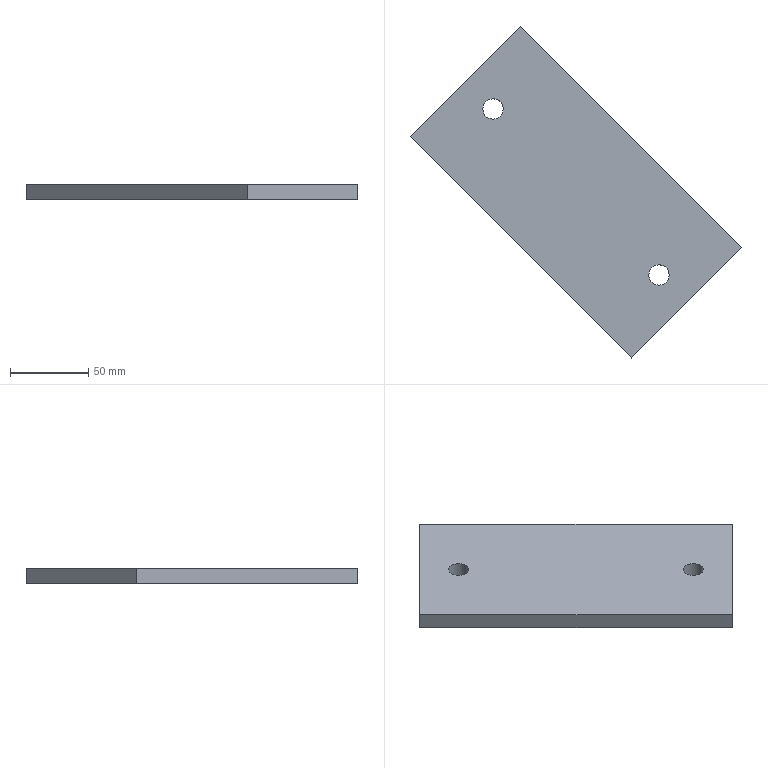Component | NX | CONN_FRAME_CONN_PLATE | 1 solid | 8 faces | box 212.13 x 212.13 x 10 mm | volume 197345 mm3 | plane 6 | cylinder 2 | commonest cylinder face diameters 13 x2
STEP:
#1=CARTESIAN_POINT('',(0.,0.,0.));
#2=DIRECTION('',(0.,0.,1.));
#3=DIRECTION('',(1.,0.,0.));
#4=AXIS2_PLACEMENT_3D('',#1,#2,#3);
#5=CARTESIAN_POINT('',(-344.075,421.231,520.));
#6=VERTEX_POINT('',#5);
#7=CARTESIAN_POINT('',(-202.653,279.81,520.));
#8=VERTEX_POINT('',#7);
#9=CARTESIAN_POINT('',(-344.075,421.231,520.));
#10=DIRECTION('',(0.7071,-0.7071,0.));
#11=VECTOR('',#10,1.);
#12=LINE('',#9,#11);
#13=CARTESIAN_POINT('',(-344.075,421.231,530.));
#14=DIRECTION('',(0.7071,0.7071,0.));
#15=DIRECTION('',(0.,0.,-1.));
#16=AXIS2_PLACEMENT_3D('',#13,#14,#15);
#17=PLANE('',#16);
#18=CARTESIAN_POINT('',(10.,0.));
#19=DIRECTION('',(0.,-1.));
#20=VECTOR('',#19,1.);
#21=LINE('',#18,#20);
#22=(GEOMETRIC_REPRESENTATION_CONTEXT(2)PARAMETRIC_REPRESENTATION_CONTEXT()REPRESENTATION_CONTEXT('',''));
#23=DEFINITIONAL_REPRESENTATION('',(#21),#22);
#24=PCURVE('',#17,#23);
#25=CARTESIAN_POINT('',(-361.752,368.198,520.));
#26=DIRECTION('',(0.,0.,1.));
#27=DIRECTION('',(-0.7071,0.7071,0.));
#28=AXIS2_PLACEMENT_3D('',#25,#26,#27);
#29=PLANE('',#28);
#30=CARTESIAN_POINT('',(25.,-50.));
#31=DIRECTION('',(-1.,0.));
#32=VECTOR('',#31,1.);
#33=LINE('',#30,#32);
#34=(GEOMETRIC_REPRESENTATION_CONTEXT(2)PARAMETRIC_REPRESENTATION_CONTEXT()REPRESENTATION_CONTEXT('',''));
#35=DEFINITIONAL_REPRESENTATION('',(#33),#34);
#36=PCURVE('',#29,#35);
#37=SURFACE_CURVE('',#12,(#24,#36),.PCURVE_S1.);
#38=EDGE_CURVE('',#6,#8,#37,.T.);
#39=ORIENTED_EDGE('',*,*,#38,.F.);
#40=CARTESIAN_POINT('',(-344.075,421.231,530.));
#41=VERTEX_POINT('',#40);
#42=CARTESIAN_POINT('',(-344.075,421.231,530.));
#43=DIRECTION('',(0.,0.,-1.));
#44=VECTOR('',#43,1.);
#45=LINE('',#42,#44);
#46=CARTESIAN_POINT('',(0.,0.));
#47=DIRECTION('',(1.,0.));
#48=VECTOR('',#47,1.);
#49=LINE('',#46,#48);
#50=(GEOMETRIC_REPRESENTATION_CONTEXT(2)PARAMETRIC_REPRESENTATION_CONTEXT()REPRESENTATION_CONTEXT('',''));
#51=DEFINITIONAL_REPRESENTATION('',(#49),#50);
#52=PCURVE('',#17,#51);
#53=CARTESIAN_POINT('',(-414.785,350.52,530.));
#54=DIRECTION('',(-0.7071,0.7071,0.));
#55=DIRECTION('',(0.,0.,-1.));
#56=AXIS2_PLACEMENT_3D('',#53,#54,#55);
#57=PLANE('',#56);
#58=CARTESIAN_POINT('',(0.,-100.));
#59=DIRECTION('',(1.,0.));
#60=VECTOR('',#59,1.);
#61=LINE('',#58,#60);
#62=(GEOMETRIC_REPRESENTATION_CONTEXT(2)PARAMETRIC_REPRESENTATION_CONTEXT()REPRESENTATION_CONTEXT('',''));
#63=DEFINITIONAL_REPRESENTATION('',(#61),#62);
#64=PCURVE('',#57,#63);
#65=SURFACE_CURVE('',#45,(#52,#64),.PCURVE_S1.);
#66=EDGE_CURVE('',#41,#6,#65,.T.);
#67=ORIENTED_EDGE('',*,*,#66,.F.);
#68=CARTESIAN_POINT('',(-202.653,279.81,530.));
#69=VERTEX_POINT('',#68);
#70=CARTESIAN_POINT('',(-344.075,421.231,530.));
#71=DIRECTION('',(0.7071,-0.7071,0.));
#72=VECTOR('',#71,1.);
#73=LINE('',#70,#72);
#74=CARTESIAN_POINT('',(0.,0.));
#75=DIRECTION('',(0.,-1.));
#76=VECTOR('',#75,1.);
#77=LINE('',#74,#76);
#78=(GEOMETRIC_REPRESENTATION_CONTEXT(2)PARAMETRIC_REPRESENTATION_CONTEXT()REPRESENTATION_CONTEXT('',''));
#79=DEFINITIONAL_REPRESENTATION('',(#77),#78);
#80=PCURVE('',#17,#79);
#81=CARTESIAN_POINT('',(-361.752,368.198,530.));
#82=DIRECTION('',(0.,0.,1.));
#83=DIRECTION('',(-0.7071,0.7071,0.));
#84=AXIS2_PLACEMENT_3D('',#81,#82,#83);
#85=PLANE('',#84);
#86=CARTESIAN_POINT('',(25.,-50.));
#87=DIRECTION('',(-1.,0.));
#88=VECTOR('',#87,1.);
#89=LINE('',#86,#88);
#90=(GEOMETRIC_REPRESENTATION_CONTEXT(2)PARAMETRIC_REPRESENTATION_CONTEXT()REPRESENTATION_CONTEXT('',''));
#91=DEFINITIONAL_REPRESENTATION('',(#89),#90);
#92=PCURVE('',#85,#91);
#93=SURFACE_CURVE('',#73,(#80,#92),.PCURVE_S1.);
#94=EDGE_CURVE('',#41,#69,#93,.T.);
#95=ORIENTED_EDGE('',*,*,#94,.T.);
#96=CARTESIAN_POINT('',(-202.653,279.81,530.));
#97=DIRECTION('',(0.,0.,-1.));
#98=VECTOR('',#97,1.);
#99=LINE('',#96,#98);
#100=CARTESIAN_POINT('',(0.,-200.));
#101=DIRECTION('',(1.,0.));
#102=VECTOR('',#101,1.);
#103=LINE('',#100,#102);
#104=(GEOMETRIC_REPRESENTATION_CONTEXT(2)PARAMETRIC_REPRESENTATION_CONTEXT()REPRESENTATION_CONTEXT('',''));
#105=DEFINITIONAL_REPRESENTATION('',(#103),#104);
#106=PCURVE('',#17,#105);
#107=CARTESIAN_POINT('',(-202.653,279.81,530.));
#108=DIRECTION('',(0.7071,-0.7071,0.));
#109=DIRECTION('',(0.,0.,1.));
#110=AXIS2_PLACEMENT_3D('',#107,#108,#109);
#111=PLANE('',#110);
#112=CARTESIAN_POINT('',(0.,0.));
#113=DIRECTION('',(-1.,0.));
#114=VECTOR('',#113,1.);
#115=LINE('',#112,#114);
#116=(GEOMETRIC_REPRESENTATION_CONTEXT(2)PARAMETRIC_REPRESENTATION_CONTEXT()REPRESENTATION_CONTEXT('',''));
#117=DEFINITIONAL_REPRESENTATION('',(#115),#116);
#118=PCURVE('',#111,#117);
#119=SURFACE_CURVE('',#99,(#106,#118),.PCURVE_S1.);
#120=EDGE_CURVE('',#69,#8,#119,.T.);
#121=ORIENTED_EDGE('',*,*,#120,.T.);
#122=EDGE_LOOP('',(#39,#67,#95,#121));
#123=FACE_BOUND('',#122,.T.);
#124=ADVANCED_FACE('',(#123),#17,.T.);
#125=CARTESIAN_POINT('',(-273.364,209.099,520.));
#126=VERTEX_POINT('',#125);
#127=CARTESIAN_POINT('',(-202.653,279.81,520.));
#128=DIRECTION('',(-0.7071,-0.7071,0.));
#129=VECTOR('',#128,1.);
#130=LINE('',#127,#129);
#131=CARTESIAN_POINT('',(-10.,0.));
#132=DIRECTION('',(0.,1.));
#133=VECTOR('',#132,1.);
#134=LINE('',#131,#133);
#135=(GEOMETRIC_REPRESENTATION_CONTEXT(2)PARAMETRIC_REPRESENTATION_CONTEXT()REPRESENTATION_CONTEXT('',''));
#136=DEFINITIONAL_REPRESENTATION('',(#134),#135);
#137=PCURVE('',#111,#136);
#138=CARTESIAN_POINT('',(-175.,-50.));
#139=DIRECTION('',(0.,1.));
#140=VECTOR('',#139,1.);
#141=LINE('',#138,#140);
#142=(GEOMETRIC_REPRESENTATION_CONTEXT(2)PARAMETRIC_REPRESENTATION_CONTEXT()REPRESENTATION_CONTEXT('',''));
#143=DEFINITIONAL_REPRESENTATION('',(#141),#142);
#144=PCURVE('',#29,#143);
#145=SURFACE_CURVE('',#130,(#137,#144),.PCURVE_S1.);
#146=EDGE_CURVE('',#8,#126,#145,.T.);
#147=ORIENTED_EDGE('',*,*,#146,.F.);
#148=ORIENTED_EDGE('',*,*,#120,.F.);
#149=CARTESIAN_POINT('',(-273.364,209.099,530.));
#150=VERTEX_POINT('',#149);
#151=CARTESIAN_POINT('',(-202.653,279.81,530.));
#152=DIRECTION('',(-0.7071,-0.7071,0.));
#153=VECTOR('',#152,1.);
#154=LINE('',#151,#153);
#155=CARTESIAN_POINT('',(0.,0.));
#156=DIRECTION('',(0.,1.));
#157=VECTOR('',#156,1.);
#158=LINE('',#155,#157);
#159=(GEOMETRIC_REPRESENTATION_CONTEXT(2)PARAMETRIC_REPRESENTATION_CONTEXT()REPRESENTATION_CONTEXT('',''));
#160=DEFINITIONAL_REPRESENTATION('',(#158),#159);
#161=PCURVE('',#111,#160);
#162=CARTESIAN_POINT('',(-175.,-50.));
#163=DIRECTION('',(0.,1.));
#164=VECTOR('',#163,1.);
#165=LINE('',#162,#164);
#166=(GEOMETRIC_REPRESENTATION_CONTEXT(2)PARAMETRIC_REPRESENTATION_CONTEXT()REPRESENTATION_CONTEXT('',''));
#167=DEFINITIONAL_REPRESENTATION('',(#165),#166);
#168=PCURVE('',#85,#167);
#169=SURFACE_CURVE('',#154,(#161,#168),.PCURVE_S1.);
#170=EDGE_CURVE('',#69,#150,#169,.T.);
#171=ORIENTED_EDGE('',*,*,#170,.T.);
#172=CARTESIAN_POINT('',(-273.364,209.099,530.));
#173=DIRECTION('',(0.,0.,-1.));
#174=VECTOR('',#173,1.);
#175=LINE('',#172,#174);
#176=CARTESIAN_POINT('',(0.,100.));
#177=DIRECTION('',(-1.,0.));
#178=VECTOR('',#177,1.);
#179=LINE('',#176,#178);
#180=(GEOMETRIC_REPRESENTATION_CONTEXT(2)PARAMETRIC_REPRESENTATION_CONTEXT()REPRESENTATION_CONTEXT('',''));
#181=DEFINITIONAL_REPRESENTATION('',(#179),#180);
#182=PCURVE('',#111,#181);
#183=CARTESIAN_POINT('',(-273.364,209.099,530.));
#184=DIRECTION('',(-0.7071,-0.7071,0.));
#185=DIRECTION('',(0.,0.,1.));
#186=AXIS2_PLACEMENT_3D('',#183,#184,#185);
#187=PLANE('',#186);
#188=CARTESIAN_POINT('',(0.,0.));
#189=DIRECTION('',(-1.,0.));
#190=VECTOR('',#189,1.);
#191=LINE('',#188,#190);
#192=(GEOMETRIC_REPRESENTATION_CONTEXT(2)PARAMETRIC_REPRESENTATION_CONTEXT()REPRESENTATION_CONTEXT('',''));
#193=DEFINITIONAL_REPRESENTATION('',(#191),#192);
#194=PCURVE('',#187,#193);
#195=SURFACE_CURVE('',#175,(#182,#194),.PCURVE_S1.);
#196=EDGE_CURVE('',#150,#126,#195,.T.);
#197=ORIENTED_EDGE('',*,*,#196,.T.);
#198=EDGE_LOOP('',(#147,#148,#171,#197));
#199=FACE_BOUND('',#198,.T.);
#200=ADVANCED_FACE('',(#199),#111,.T.);
#201=CARTESIAN_POINT('',(-414.785,350.52,520.));
#202=VERTEX_POINT('',#201);
#203=CARTESIAN_POINT('',(-273.364,209.099,520.));
#204=DIRECTION('',(-0.7071,0.7071,0.));
#205=VECTOR('',#204,1.);
#206=LINE('',#203,#205);
#207=CARTESIAN_POINT('',(-10.,0.));
#208=DIRECTION('',(0.,1.));
#209=VECTOR('',#208,1.);
#210=LINE('',#207,#209);
#211=(GEOMETRIC_REPRESENTATION_CONTEXT(2)PARAMETRIC_REPRESENTATION_CONTEXT()REPRESENTATION_CONTEXT('',''));
#212=DEFINITIONAL_REPRESENTATION('',(#210),#211);
#213=PCURVE('',#187,#212);
#214=CARTESIAN_POINT('',(-175.,50.));
#215=DIRECTION('',(1.,0.));
#216=VECTOR('',#215,1.);
#217=LINE('',#214,#216);
#218=(GEOMETRIC_REPRESENTATION_CONTEXT(2)PARAMETRIC_REPRESENTATION_CONTEXT()REPRESENTATION_CONTEXT('',''));
#219=DEFINITIONAL_REPRESENTATION('',(#217),#218);
#220=PCURVE('',#29,#219);
#221=SURFACE_CURVE('',#206,(#213,#220),.PCURVE_S1.);
#222=EDGE_CURVE('',#126,#202,#221,.T.);
#223=ORIENTED_EDGE('',*,*,#222,.F.);
#224=ORIENTED_EDGE('',*,*,#196,.F.);
#225=CARTESIAN_POINT('',(-414.785,350.52,530.));
#226=VERTEX_POINT('',#225);
#227=CARTESIAN_POINT('',(-273.364,209.099,530.));
#228=DIRECTION('',(-0.7071,0.7071,0.));
#229=VECTOR('',#228,1.);
#230=LINE('',#227,#229);
#231=CARTESIAN_POINT('',(0.,0.));
#232=DIRECTION('',(0.,1.));
#233=VECTOR('',#232,1.);
#234=LINE('',#231,#233);
#235=(GEOMETRIC_REPRESENTATION_CONTEXT(2)PARAMETRIC_REPRESENTATION_CONTEXT()REPRESENTATION_CONTEXT('',''));
#236=DEFINITIONAL_REPRESENTATION('',(#234),#235);
#237=PCURVE('',#187,#236);
#238=CARTESIAN_POINT('',(-175.,50.));
#239=DIRECTION('',(1.,0.));
#240=VECTOR('',#239,1.);
#241=LINE('',#238,#240);
#242=(GEOMETRIC_REPRESENTATION_CONTEXT(2)PARAMETRIC_REPRESENTATION_CONTEXT()REPRESENTATION_CONTEXT('',''));
#243=DEFINITIONAL_REPRESENTATION('',(#241),#242);
#244=PCURVE('',#85,#243);
#245=SURFACE_CURVE('',#230,(#237,#244),.PCURVE_S1.);
#246=EDGE_CURVE('',#150,#226,#245,.T.);
#247=ORIENTED_EDGE('',*,*,#246,.T.);
#248=CARTESIAN_POINT('',(-414.785,350.52,530.));
#249=DIRECTION('',(0.,0.,-1.));
#250=VECTOR('',#249,1.);
#251=LINE('',#248,#250);
#252=CARTESIAN_POINT('',(0.,200.));
#253=DIRECTION('',(-1.,0.));
#254=VECTOR('',#253,1.);
#255=LINE('',#252,#254);
#256=(GEOMETRIC_REPRESENTATION_CONTEXT(2)PARAMETRIC_REPRESENTATION_CONTEXT()REPRESENTATION_CONTEXT('',''));
#257=DEFINITIONAL_REPRESENTATION('',(#255),#256);
#258=PCURVE('',#187,#257);
#259=CARTESIAN_POINT('',(0.,0.));
#260=DIRECTION('',(1.,0.));
#261=VECTOR('',#260,1.);
#262=LINE('',#259,#261);
#263=(GEOMETRIC_REPRESENTATION_CONTEXT(2)PARAMETRIC_REPRESENTATION_CONTEXT()REPRESENTATION_CONTEXT('',''));
#264=DEFINITIONAL_REPRESENTATION('',(#262),#263);
#265=PCURVE('',#57,#264);
#266=SURFACE_CURVE('',#251,(#258,#265),.PCURVE_S1.);
#267=EDGE_CURVE('',#226,#202,#266,.T.);
#268=ORIENTED_EDGE('',*,*,#267,.T.);
#269=EDGE_LOOP('',(#223,#224,#247,#268));
#270=FACE_BOUND('',#269,.T.);
#271=ADVANCED_FACE('',(#270),#187,.T.);
#272=CARTESIAN_POINT('',(-357.156,363.602,530.));
#273=VERTEX_POINT('',#272);
#274=CARTESIAN_POINT('',(-361.752,368.198,530.));
#275=DIRECTION('',(0.,0.,1.));
#276=DIRECTION('',(0.7071,-0.7071,0.));
#277=AXIS2_PLACEMENT_3D('',#274,#275,#276);
#278=CIRCLE('',#277,6.5);
#279=CARTESIAN_POINT('',(-361.752,368.198,530.));
#280=DIRECTION('',(0.,0.,-1.));
#281=DIRECTION('',(0.7071,-0.7071,0.));
#282=AXIS2_PLACEMENT_3D('',#279,#280,#281);
#283=CYLINDRICAL_SURFACE('',#282,6.5);
#284=CARTESIAN_POINT('',(6.283,0.));
#285=DIRECTION('',(-1.,0.));
#286=VECTOR('',#285,1.);
#287=LINE('',#284,#286);
#288=(GEOMETRIC_REPRESENTATION_CONTEXT(2)PARAMETRIC_REPRESENTATION_CONTEXT()REPRESENTATION_CONTEXT('',''));
#289=DEFINITIONAL_REPRESENTATION('',(#287),#288);
#290=PCURVE('',#283,#289);
#291=CARTESIAN_POINT('',(0.,0.));
#292=DIRECTION('',(-1.,-0.));
#293=AXIS2_PLACEMENT_2D('',#291,#292);
#294=CIRCLE('',#293,6.5);
#295=(GEOMETRIC_REPRESENTATION_CONTEXT(2)PARAMETRIC_REPRESENTATION_CONTEXT()REPRESENTATION_CONTEXT('',''));
#296=DEFINITIONAL_REPRESENTATION('',(#294),#295);
#297=PCURVE('',#85,#296);
#298=SURFACE_CURVE('',#278,(#290,#297),.PCURVE_S1.);
#299=EDGE_CURVE('',#273,#273,#298,.T.);
#300=ORIENTED_EDGE('',*,*,#299,.F.);
#301=CARTESIAN_POINT('',(-357.156,363.602,520.));
#302=VERTEX_POINT('',#301);
#303=CARTESIAN_POINT('',(-357.156,363.602,530.));
#304=CARTESIAN_POINT('',(-357.156,363.602,520.));
#305=B_SPLINE_CURVE_WITH_KNOTS('',1,(#303,#304),.UNSPECIFIED.,.F.,.F.,(2,2),(0.,10.),.PIECEWISE_BEZIER_KNOTS.);
#306=CARTESIAN_POINT('',(6.283,0.));
#307=DIRECTION('',(0.,1.));
#308=VECTOR('',#307,1.);
#309=LINE('',#306,#308);
#310=(GEOMETRIC_REPRESENTATION_CONTEXT(2)PARAMETRIC_REPRESENTATION_CONTEXT()REPRESENTATION_CONTEXT('',''));
#311=DEFINITIONAL_REPRESENTATION('',(#309),#310);
#312=PCURVE('',#283,#311);
#313=CARTESIAN_POINT('',(0.,0.));
#314=DIRECTION('',(0.,1.));
#315=VECTOR('',#314,1.);
#316=LINE('',#313,#315);
#317=(GEOMETRIC_REPRESENTATION_CONTEXT(2)PARAMETRIC_REPRESENTATION_CONTEXT()REPRESENTATION_CONTEXT('',''));
#318=DEFINITIONAL_REPRESENTATION('',(#316),#317);
#319=PCURVE('',#283,#318);
#320=SEAM_CURVE('',#305,(#312,#319),.PCURVE_S1.);
#321=EDGE_CURVE('',#273,#302,#320,.T.);
#322=ORIENTED_EDGE('',*,*,#321,.T.);
#323=CARTESIAN_POINT('',(-361.752,368.198,520.));
#324=DIRECTION('',(0.,0.,1.));
#325=DIRECTION('',(0.7071,-0.7071,0.));
#326=AXIS2_PLACEMENT_3D('',#323,#324,#325);
#327=CIRCLE('',#326,6.5);
#328=CARTESIAN_POINT('',(6.283,10.));
#329=DIRECTION('',(-1.,0.));
#330=VECTOR('',#329,1.);
#331=LINE('',#328,#330);
#332=(GEOMETRIC_REPRESENTATION_CONTEXT(2)PARAMETRIC_REPRESENTATION_CONTEXT()REPRESENTATION_CONTEXT('',''));
#333=DEFINITIONAL_REPRESENTATION('',(#331),#332);
#334=PCURVE('',#283,#333);
#335=CARTESIAN_POINT('',(0.,0.));
#336=DIRECTION('',(-1.,-0.));
#337=AXIS2_PLACEMENT_2D('',#335,#336);
#338=CIRCLE('',#337,6.5);
#339=(GEOMETRIC_REPRESENTATION_CONTEXT(2)PARAMETRIC_REPRESENTATION_CONTEXT()REPRESENTATION_CONTEXT('',''));
#340=DEFINITIONAL_REPRESENTATION('',(#338),#339);
#341=PCURVE('',#29,#340);
#342=SURFACE_CURVE('',#327,(#334,#341),.PCURVE_S1.);
#343=EDGE_CURVE('',#302,#302,#342,.T.);
#344=ORIENTED_EDGE('',*,*,#343,.T.);
#345=ORIENTED_EDGE('',*,*,#321,.F.);
#346=EDGE_LOOP('',(#300,#322,#344,#345));
#347=FACE_BOUND('',#346,.F.);
#348=ADVANCED_FACE('',(#347),#283,.F.);
#349=CARTESIAN_POINT('',(-414.785,350.52,520.));
#350=DIRECTION('',(0.7071,0.7071,0.));
#351=VECTOR('',#350,1.);
#352=LINE('',#349,#351);
#353=CARTESIAN_POINT('',(10.,0.));
#354=DIRECTION('',(0.,-1.));
#355=VECTOR('',#354,1.);
#356=LINE('',#353,#355);
#357=(GEOMETRIC_REPRESENTATION_CONTEXT(2)PARAMETRIC_REPRESENTATION_CONTEXT()REPRESENTATION_CONTEXT('',''));
#358=DEFINITIONAL_REPRESENTATION('',(#356),#357);
#359=PCURVE('',#57,#358);
#360=CARTESIAN_POINT('',(25.,50.));
#361=DIRECTION('',(0.,-1.));
#362=VECTOR('',#361,1.);
#363=LINE('',#360,#362);
#364=(GEOMETRIC_REPRESENTATION_CONTEXT(2)PARAMETRIC_REPRESENTATION_CONTEXT()REPRESENTATION_CONTEXT('',''));
#365=DEFINITIONAL_REPRESENTATION('',(#363),#364);
#366=PCURVE('',#29,#365);
#367=SURFACE_CURVE('',#352,(#359,#366),.PCURVE_S1.);
#368=EDGE_CURVE('',#202,#6,#367,.T.);
#369=ORIENTED_EDGE('',*,*,#368,.F.);
#370=ORIENTED_EDGE('',*,*,#267,.F.);
#371=CARTESIAN_POINT('',(-414.785,350.52,530.));
#372=DIRECTION('',(0.7071,0.7071,0.));
#373=VECTOR('',#372,1.);
#374=LINE('',#371,#373);
#375=CARTESIAN_POINT('',(0.,0.));
#376=DIRECTION('',(0.,-1.));
#377=VECTOR('',#376,1.);
#378=LINE('',#375,#377);
#379=(GEOMETRIC_REPRESENTATION_CONTEXT(2)PARAMETRIC_REPRESENTATION_CONTEXT()REPRESENTATION_CONTEXT('',''));
#380=DEFINITIONAL_REPRESENTATION('',(#378),#379);
#381=PCURVE('',#57,#380);
#382=CARTESIAN_POINT('',(25.,50.));
#383=DIRECTION('',(0.,-1.));
#384=VECTOR('',#383,1.);
#385=LINE('',#382,#384);
#386=(GEOMETRIC_REPRESENTATION_CONTEXT(2)PARAMETRIC_REPRESENTATION_CONTEXT()REPRESENTATION_CONTEXT('',''));
#387=DEFINITIONAL_REPRESENTATION('',(#385),#386);
#388=PCURVE('',#85,#387);
#389=SURFACE_CURVE('',#374,(#381,#388),.PCURVE_S1.);
#390=EDGE_CURVE('',#226,#41,#389,.T.);
#391=ORIENTED_EDGE('',*,*,#390,.T.);
#392=ORIENTED_EDGE('',*,*,#66,.T.);
#393=EDGE_LOOP('',(#369,#370,#391,#392));
#394=FACE_BOUND('',#393,.T.);
#395=ADVANCED_FACE('',(#394),#57,.T.);
#396=CARTESIAN_POINT('',(-260.283,266.728,530.));
#397=VERTEX_POINT('',#396);
#398=CARTESIAN_POINT('',(-255.686,262.132,530.));
#399=DIRECTION('',(0.,0.,-1.));
#400=DIRECTION('',(-0.7071,0.7071,0.));
#401=AXIS2_PLACEMENT_3D('',#398,#399,#400);
#402=CIRCLE('',#401,6.5);
#403=CARTESIAN_POINT('',(-255.686,262.132,530.));
#404=DIRECTION('',(0.,0.,-1.));
#405=DIRECTION('',(0.7071,-0.7071,0.));
#406=AXIS2_PLACEMENT_3D('',#403,#404,#405);
#407=CYLINDRICAL_SURFACE('',#406,6.5);
#408=CARTESIAN_POINT('',(3.142,0.));
#409=DIRECTION('',(1.,0.));
#410=VECTOR('',#409,1.);
#411=LINE('',#408,#410);
#412=(GEOMETRIC_REPRESENTATION_CONTEXT(2)PARAMETRIC_REPRESENTATION_CONTEXT()REPRESENTATION_CONTEXT('',''));
#413=DEFINITIONAL_REPRESENTATION('',(#411),#412);
#414=PCURVE('',#407,#413);
#415=CARTESIAN_POINT('',(-143.5,-0.));
#416=CARTESIAN_POINT('',(-143.5,-11.258));
#417=CARTESIAN_POINT('',(-153.25,-5.629));
#418=CARTESIAN_POINT('',(-163.,-0.));
#419=CARTESIAN_POINT('',(-153.25,5.629));
#420=CARTESIAN_POINT('',(-143.5,11.258));
#421=CARTESIAN_POINT('',(-143.5,-0.));
#422=(BOUNDED_CURVE()B_SPLINE_CURVE(2,(#415,#416,#417,#418,#419,#420,#421),.UNSPECIFIED.,.T.,.F.)B_SPLINE_CURVE_WITH_KNOTS((1,2,2,2,2,1),(-2.094,0.,2.094,4.189,6.283,8.378),.UNSPECIFIED.)CURVE()GEOMETRIC_REPRESENTATION_ITEM()RATIONAL_B_SPLINE_CURVE((1.,0.5,1.,0.5,1.,0.5,1.))REPRESENTATION_ITEM(''));
#423=(GEOMETRIC_REPRESENTATION_CONTEXT(2)PARAMETRIC_REPRESENTATION_CONTEXT()REPRESENTATION_CONTEXT('',''));
#424=DEFINITIONAL_REPRESENTATION('',(#422),#423);
#425=PCURVE('',#85,#424);
#426=SURFACE_CURVE('',#402,(#414,#425),.PCURVE_S1.);
#427=EDGE_CURVE('',#397,#397,#426,.T.);
#428=ORIENTED_EDGE('',*,*,#427,.T.);
#429=CARTESIAN_POINT('',(-260.283,266.728,520.));
#430=VERTEX_POINT('',#429);
#431=CARTESIAN_POINT('',(-260.283,266.728,530.));
#432=CARTESIAN_POINT('',(-260.283,266.728,520.));
#433=B_SPLINE_CURVE_WITH_KNOTS('',1,(#431,#432),.UNSPECIFIED.,.F.,.F.,(2,2),(0.,10.),.PIECEWISE_BEZIER_KNOTS.);
#434=CARTESIAN_POINT('',(9.425,0.));
#435=DIRECTION('',(0.,1.));
#436=VECTOR('',#435,1.);
#437=LINE('',#434,#436);
#438=(GEOMETRIC_REPRESENTATION_CONTEXT(2)PARAMETRIC_REPRESENTATION_CONTEXT()REPRESENTATION_CONTEXT('',''));
#439=DEFINITIONAL_REPRESENTATION('',(#437),#438);
#440=PCURVE('',#407,#439);
#441=CARTESIAN_POINT('',(3.142,0.));
#442=DIRECTION('',(0.,1.));
#443=VECTOR('',#442,1.);
#444=LINE('',#441,#443);
#445=(GEOMETRIC_REPRESENTATION_CONTEXT(2)PARAMETRIC_REPRESENTATION_CONTEXT()REPRESENTATION_CONTEXT('',''));
#446=DEFINITIONAL_REPRESENTATION('',(#444),#445);
#447=PCURVE('',#407,#446);
#448=SEAM_CURVE('',#433,(#440,#447),.PCURVE_S1.);
#449=EDGE_CURVE('',#397,#430,#448,.T.);
#450=ORIENTED_EDGE('',*,*,#449,.T.);
#451=CARTESIAN_POINT('',(-255.686,262.132,520.));
#452=DIRECTION('',(0.,0.,-1.));
#453=DIRECTION('',(-0.7071,0.7071,0.));
#454=AXIS2_PLACEMENT_3D('',#451,#452,#453);
#455=CIRCLE('',#454,6.5);
#456=CARTESIAN_POINT('',(3.142,10.));
#457=DIRECTION('',(1.,0.));
#458=VECTOR('',#457,1.);
#459=LINE('',#456,#458);
#460=(GEOMETRIC_REPRESENTATION_CONTEXT(2)PARAMETRIC_REPRESENTATION_CONTEXT()REPRESENTATION_CONTEXT('',''));
#461=DEFINITIONAL_REPRESENTATION('',(#459),#460);
#462=PCURVE('',#407,#461);
#463=CARTESIAN_POINT('',(-143.5,-0.));
#464=CARTESIAN_POINT('',(-143.5,-11.258));
#465=CARTESIAN_POINT('',(-153.25,-5.629));
#466=CARTESIAN_POINT('',(-163.,-0.));
#467=CARTESIAN_POINT('',(-153.25,5.629));
#468=CARTESIAN_POINT('',(-143.5,11.258));
#469=CARTESIAN_POINT('',(-143.5,-0.));
#470=(BOUNDED_CURVE()B_SPLINE_CURVE(2,(#463,#464,#465,#466,#467,#468,#469),.UNSPECIFIED.,.T.,.F.)B_SPLINE_CURVE_WITH_KNOTS((1,2,2,2,2,1),(-2.094,0.,2.094,4.189,6.283,8.378),.UNSPECIFIED.)CURVE()GEOMETRIC_REPRESENTATION_ITEM()RATIONAL_B_SPLINE_CURVE((1.,0.5,1.,0.5,1.,0.5,1.))REPRESENTATION_ITEM(''));
#471=(GEOMETRIC_REPRESENTATION_CONTEXT(2)PARAMETRIC_REPRESENTATION_CONTEXT()REPRESENTATION_CONTEXT('',''));
#472=DEFINITIONAL_REPRESENTATION('',(#470),#471);
#473=PCURVE('',#29,#472);
#474=SURFACE_CURVE('',#455,(#462,#473),.PCURVE_S1.);
#475=EDGE_CURVE('',#430,#430,#474,.T.);
#476=ORIENTED_EDGE('',*,*,#475,.F.);
#477=ORIENTED_EDGE('',*,*,#449,.F.);
#478=EDGE_LOOP('',(#428,#450,#476,#477));
#479=FACE_BOUND('',#478,.F.);
#480=ADVANCED_FACE('',(#479),#407,.F.);
#481=ORIENTED_EDGE('',*,*,#94,.F.);
#482=ORIENTED_EDGE('',*,*,#390,.F.);
#483=ORIENTED_EDGE('',*,*,#246,.F.);
#484=ORIENTED_EDGE('',*,*,#170,.F.);
#485=EDGE_LOOP('',(#481,#482,#483,#484));
#486=FACE_BOUND('',#485,.T.);
#487=ORIENTED_EDGE('',*,*,#299,.F.);
#488=EDGE_LOOP('',(#487));
#489=FACE_BOUND('',#488,.T.);
#490=ORIENTED_EDGE('',*,*,#427,.T.);
#491=EDGE_LOOP('',(#490));
#492=FACE_BOUND('',#491,.T.);
#493=ADVANCED_FACE('',(#486,#489,#492),#85,.T.);
#494=ORIENTED_EDGE('',*,*,#38,.T.);
#495=ORIENTED_EDGE('',*,*,#146,.T.);
#496=ORIENTED_EDGE('',*,*,#222,.T.);
#497=ORIENTED_EDGE('',*,*,#368,.T.);
#498=EDGE_LOOP('',(#494,#495,#496,#497));
#499=FACE_BOUND('',#498,.T.);
#500=ORIENTED_EDGE('',*,*,#343,.T.);
#501=EDGE_LOOP('',(#500));
#502=FACE_BOUND('',#501,.T.);
#503=ORIENTED_EDGE('',*,*,#475,.F.);
#504=EDGE_LOOP('',(#503));
#505=FACE_BOUND('',#504,.T.);
#506=ADVANCED_FACE('',(#499,#502,#505),#29,.F.);
#507=CLOSED_SHELL('',(#124,#200,#271,#348,#395,#480,#493,#506));
#508=MANIFOLD_SOLID_BREP('',#507);
#509=(LENGTH_UNIT()NAMED_UNIT(*)SI_UNIT(.MILLI.,.METRE.));
#510=UNCERTAINTY_MEASURE_WITH_UNIT(LENGTH_MEASURE(0.000002),#509,'','');
#511=(NAMED_UNIT(*)PLANE_ANGLE_UNIT()SI_UNIT($,.RADIAN.));
#512=(NAMED_UNIT(*)SI_UNIT($,.STERADIAN.)SOLID_ANGLE_UNIT());
#513=(GEOMETRIC_REPRESENTATION_CONTEXT(3)GLOBAL_UNCERTAINTY_ASSIGNED_CONTEXT((#510))GLOBAL_UNIT_ASSIGNED_CONTEXT((#509,#511,#512))REPRESENTATION_CONTEXT('',''));
#514=ADVANCED_BREP_SHAPE_REPRESENTATION('',(#4,#508),#513);